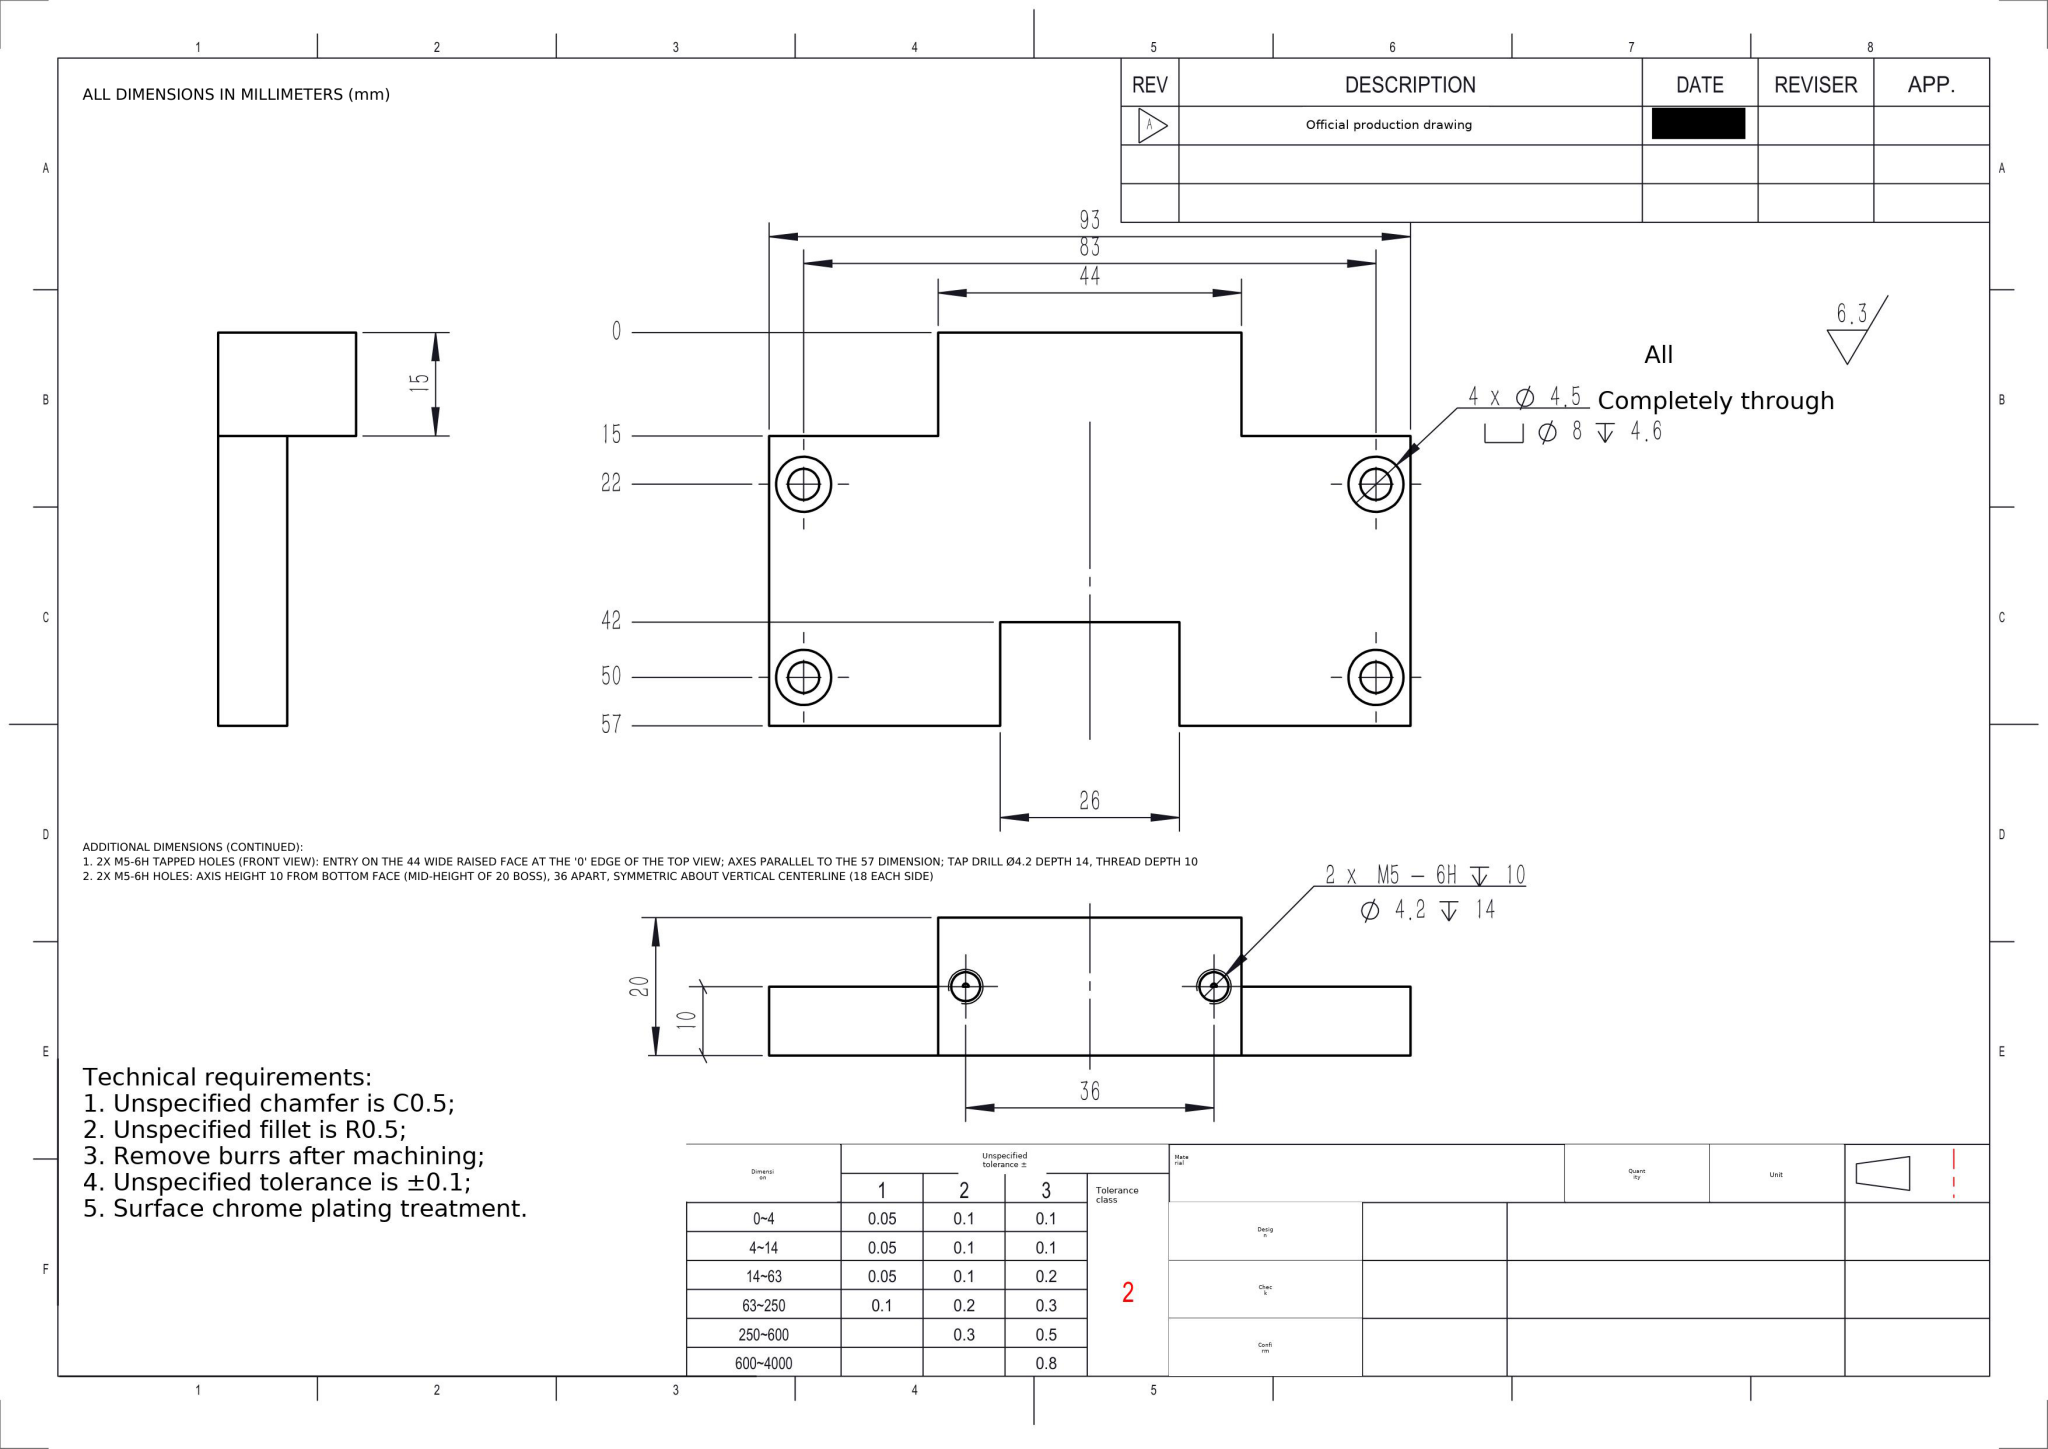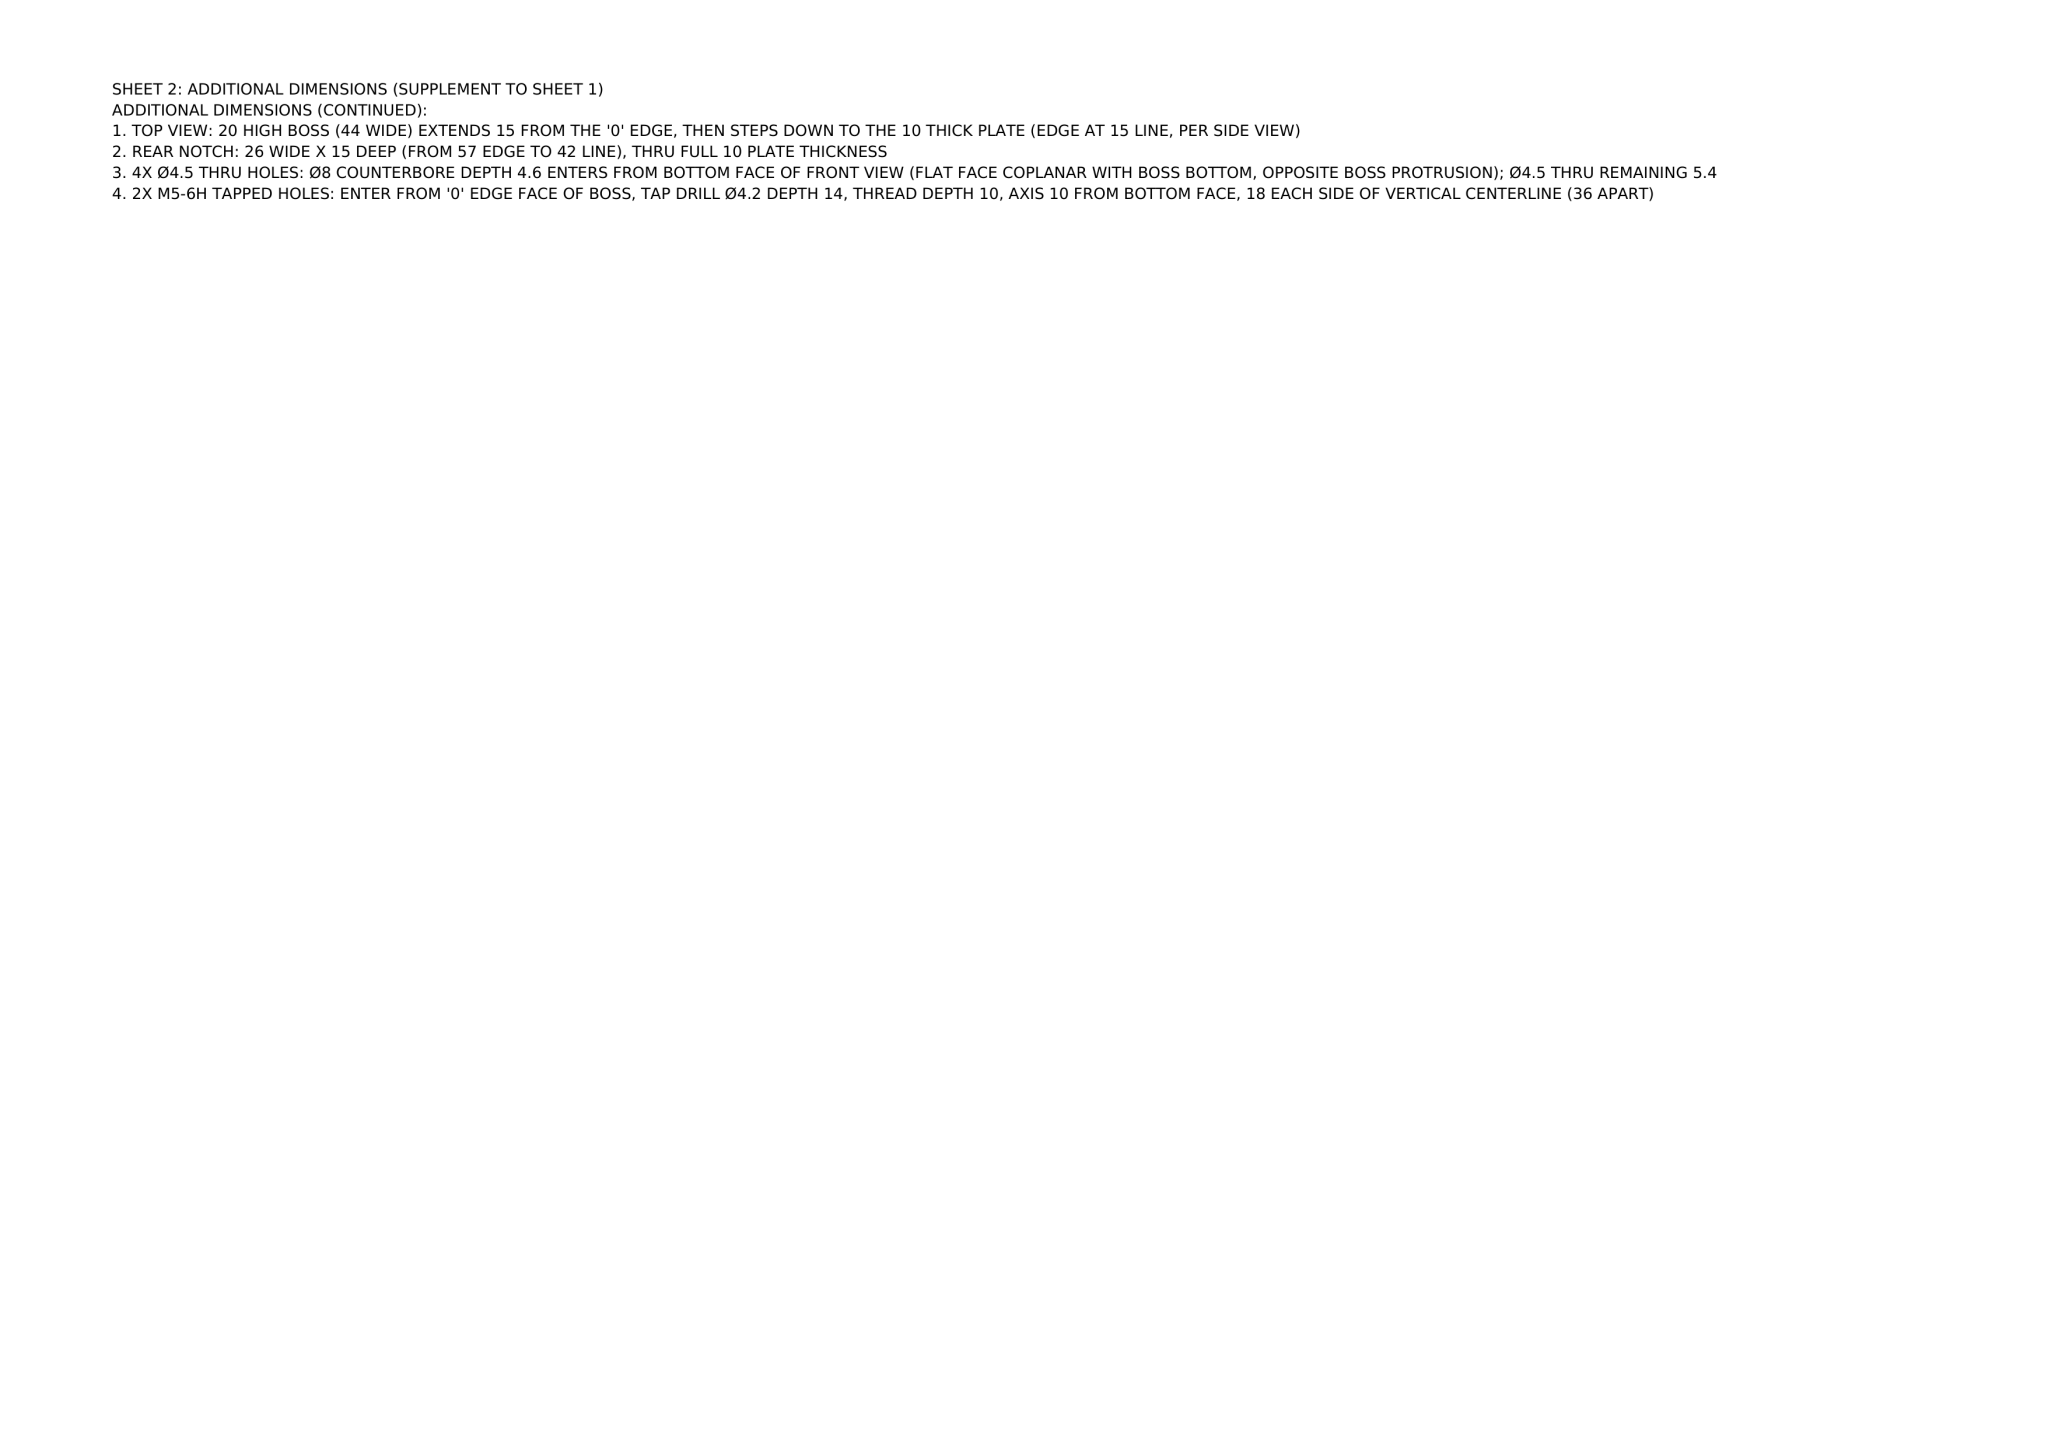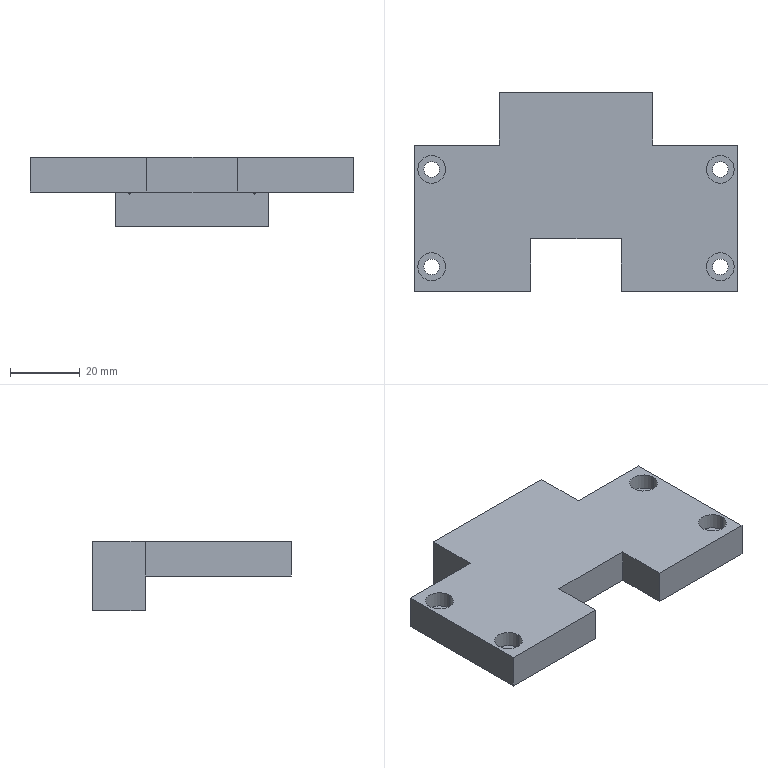Part | NX | mm | 1 solid | 44 faces | box 93 x 57 x 20 mm | volume 46692 mm3 | cylinder 20 | plane 20 | cone 4 | commonest cylinder face diameters 8 x8 4.5 x8 4.2 x4